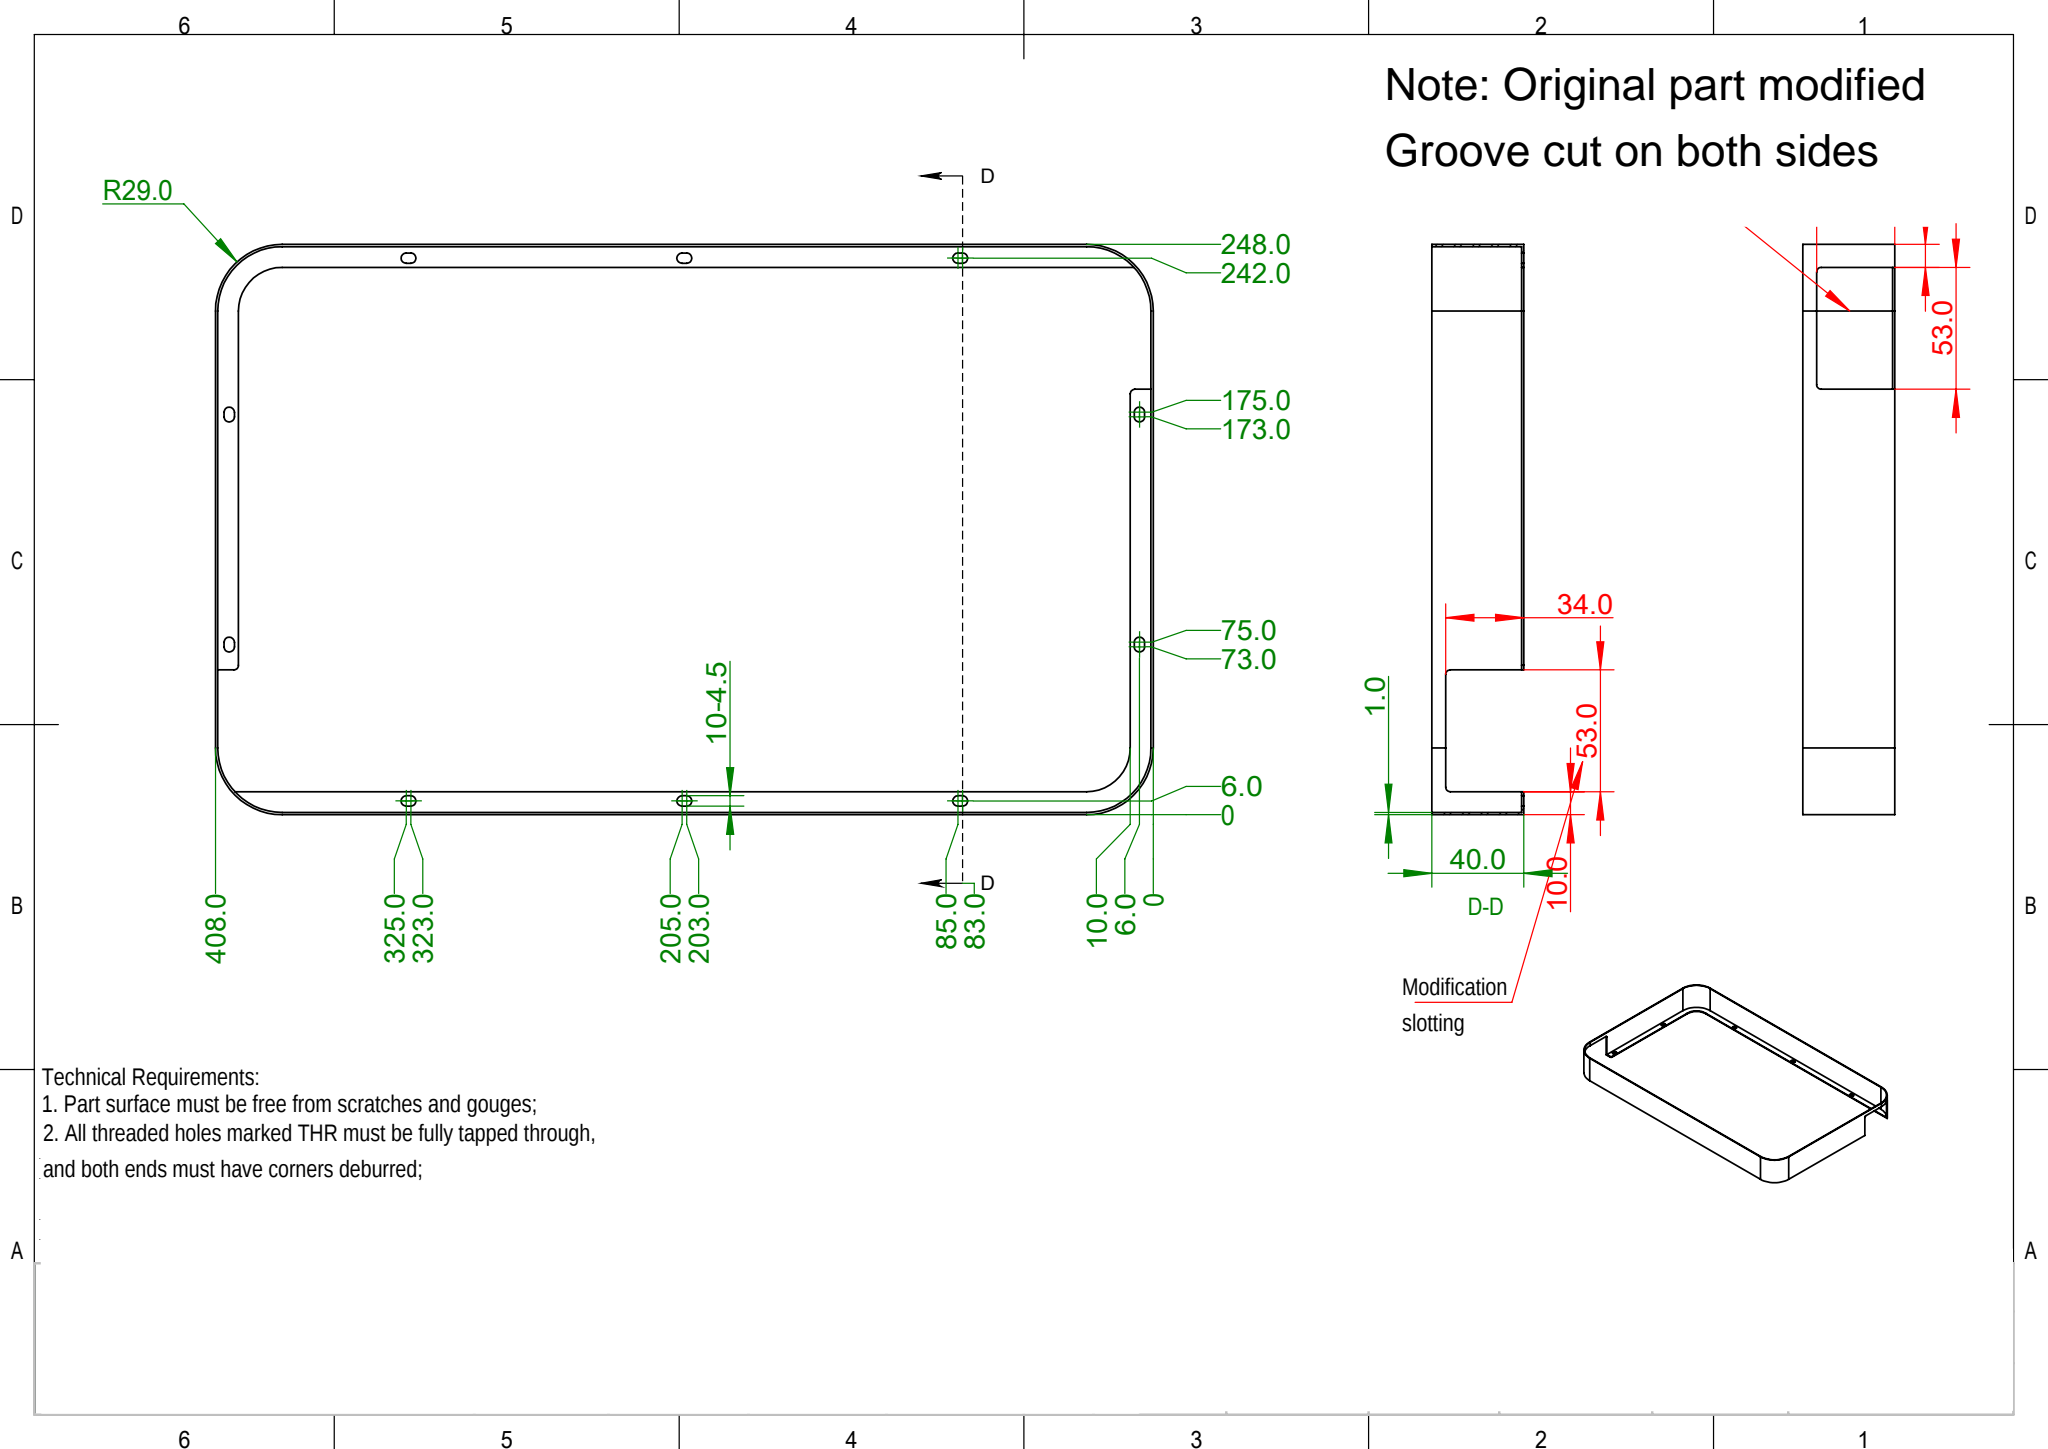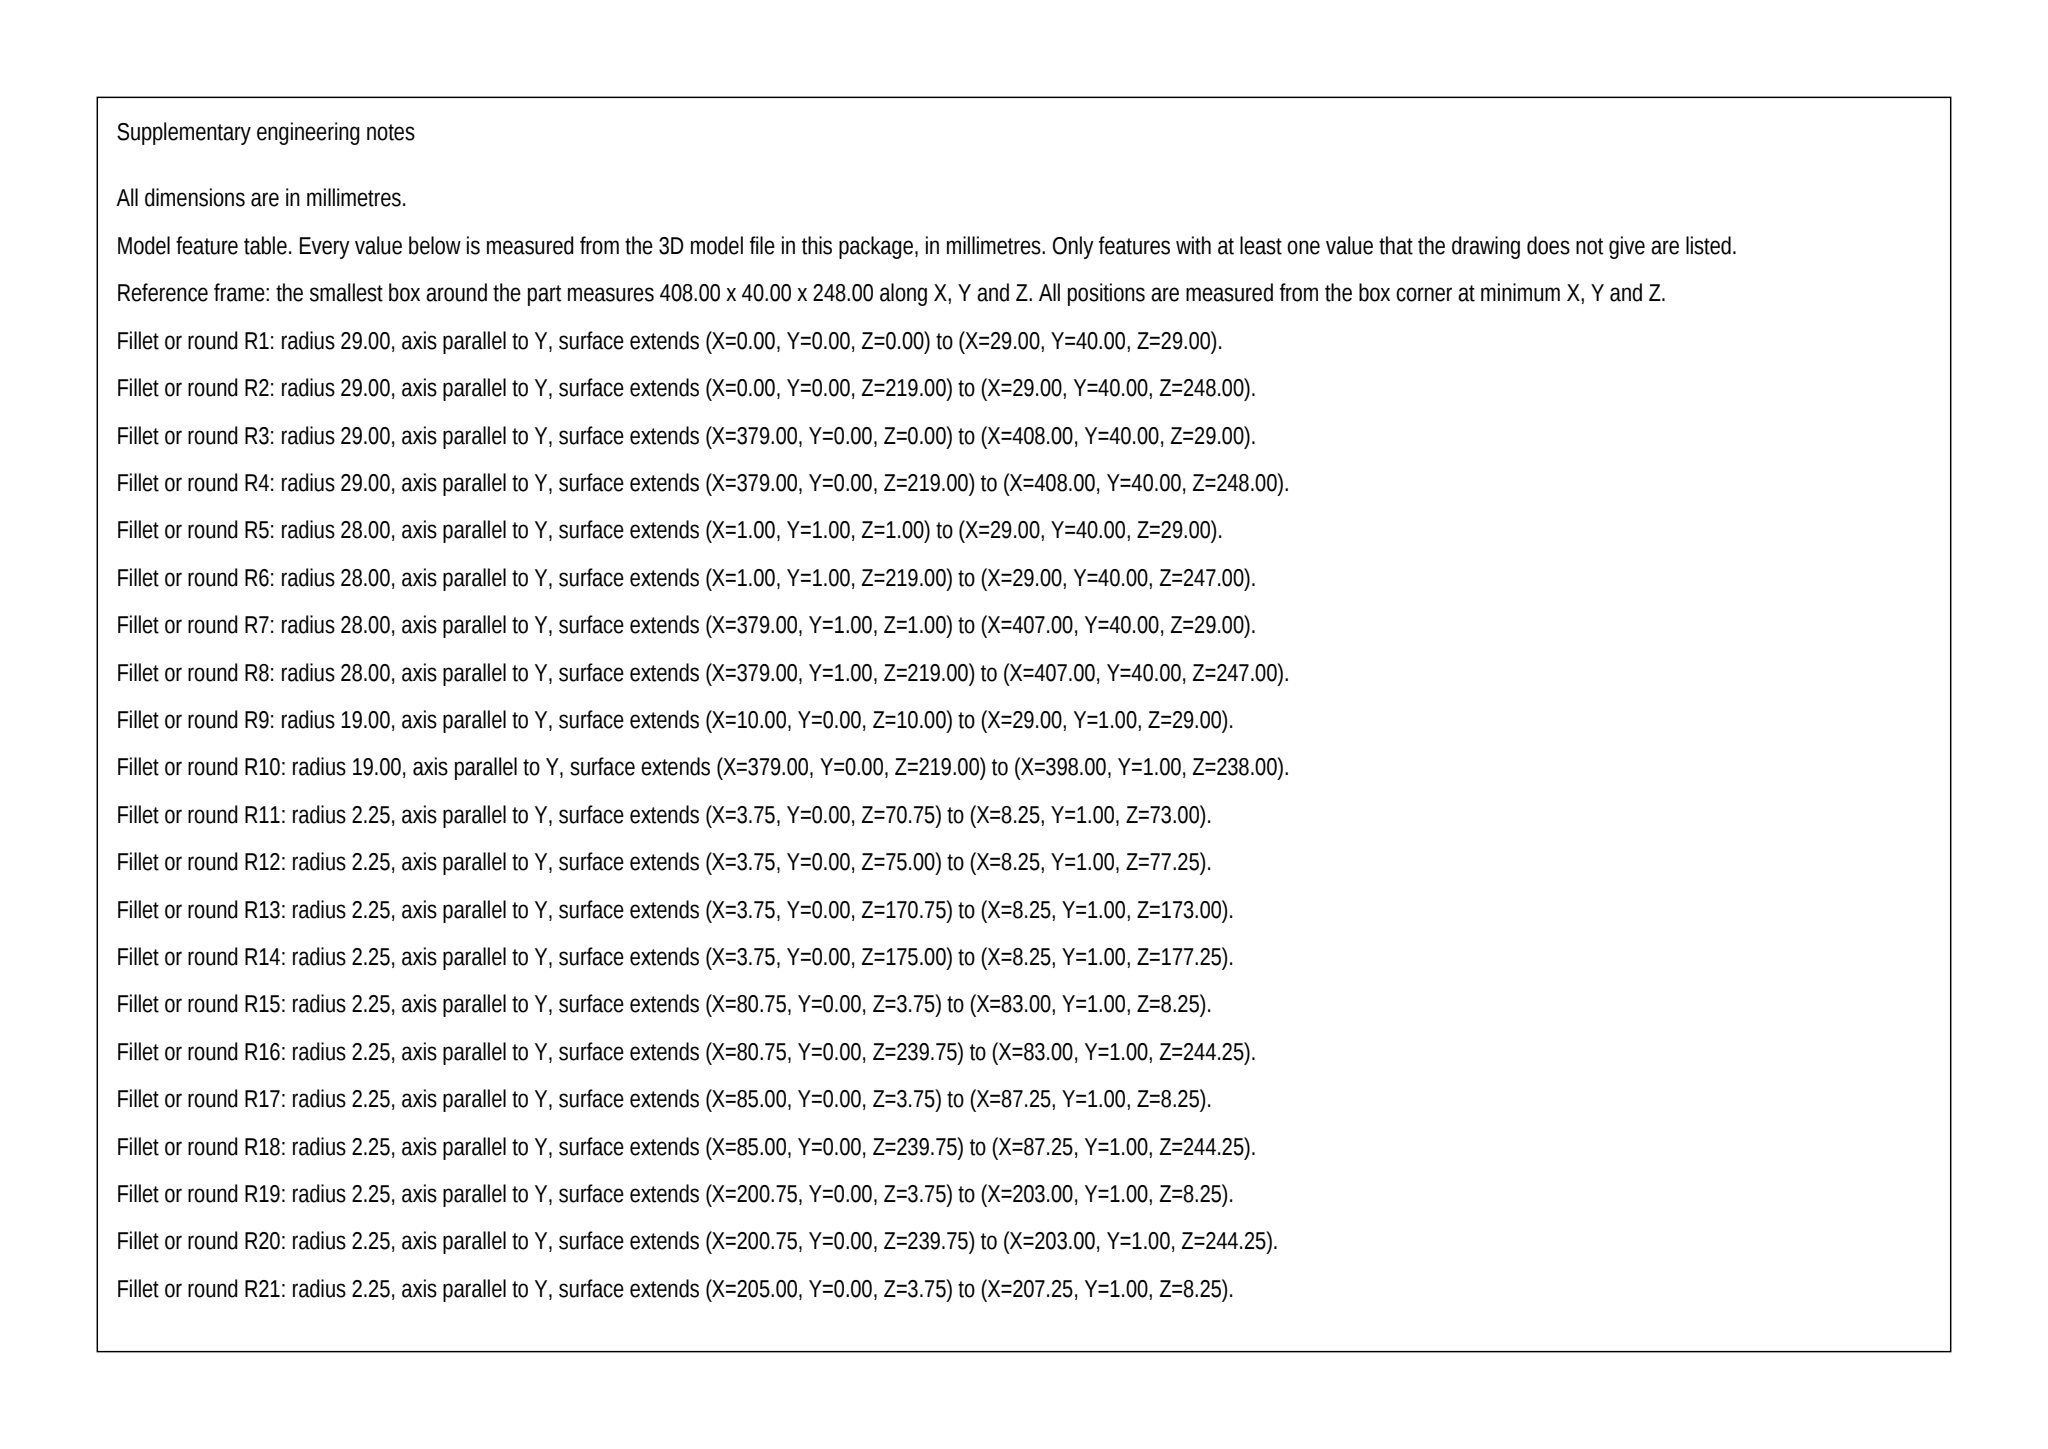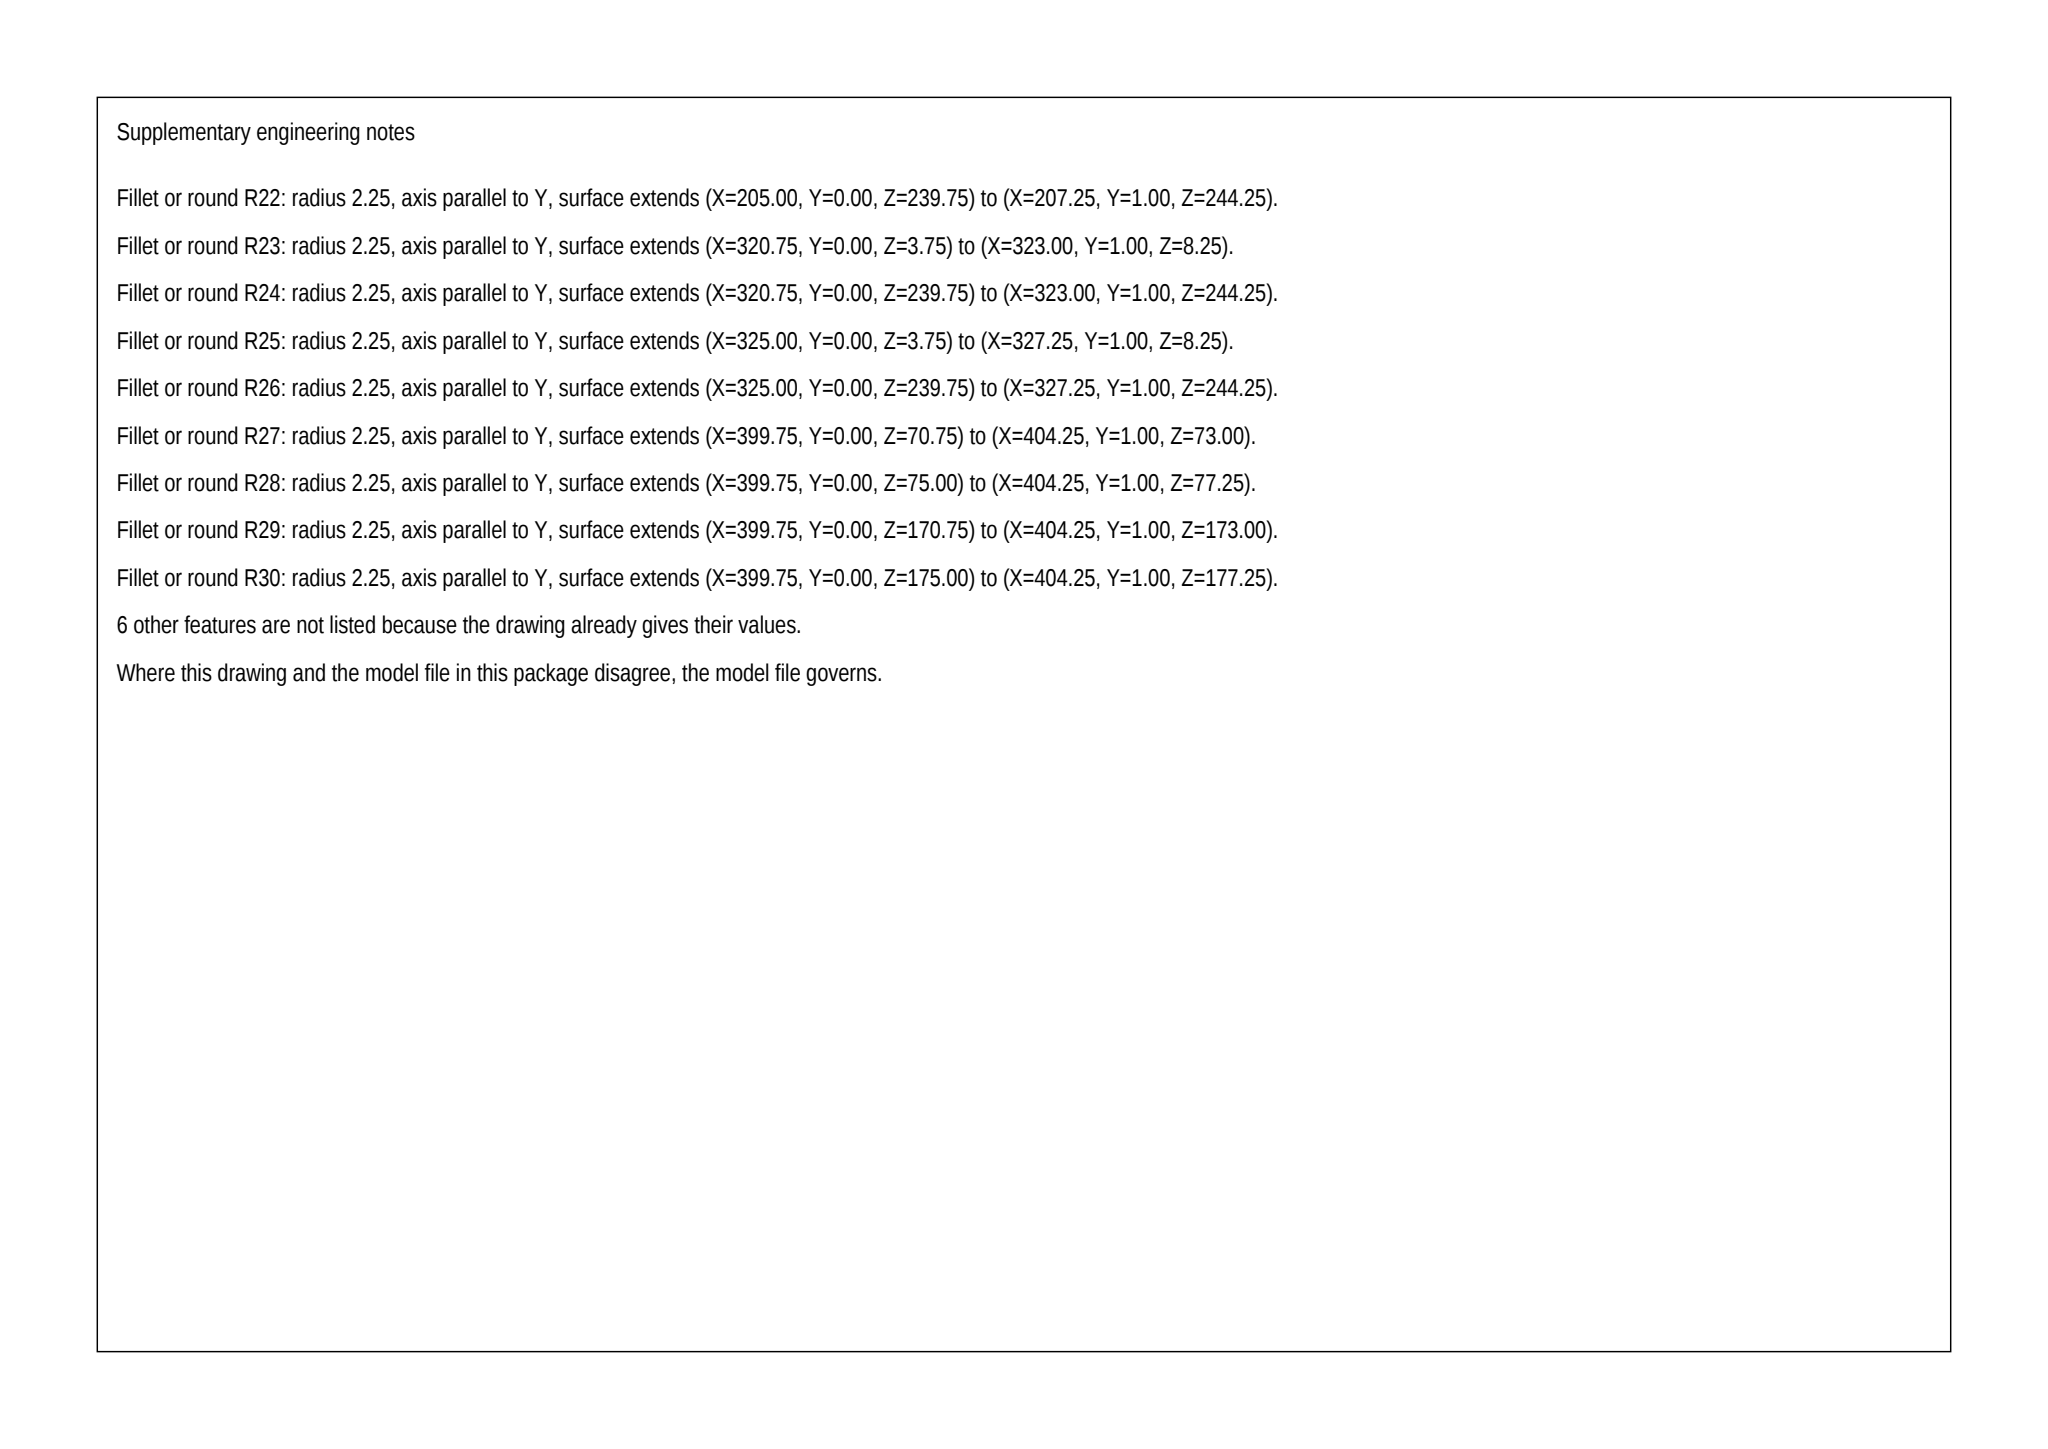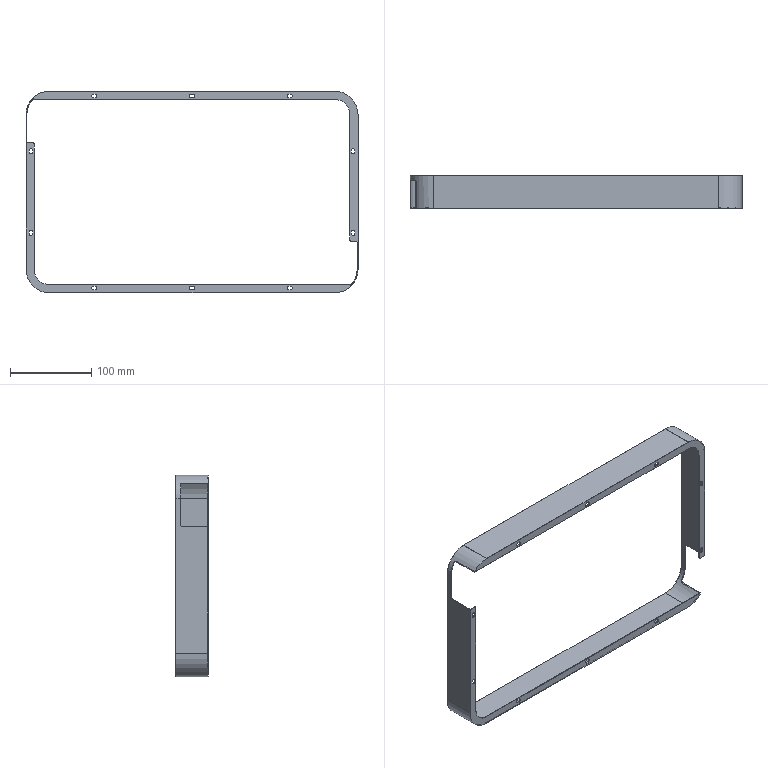Part | SolidWorks | mm | 1 solid | 81 faces | box 408 x 40 x 248 mm | volume 56418 mm3 | plane 41 | cylinder 40 | commonest cylinder face diameters 4.5 x24 4 x6 58 x4 56 x4 38 x2